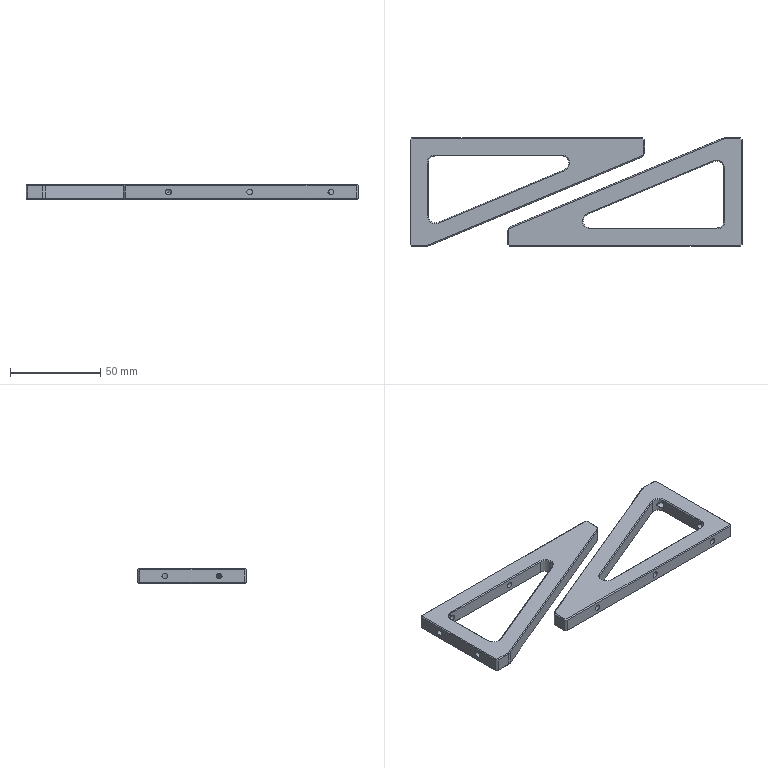CAM job | Mastercam | mm | 8 operations | part box 184.04 x 60 x 8
1. Contour (Ramp) | 6 - 6 平底刀
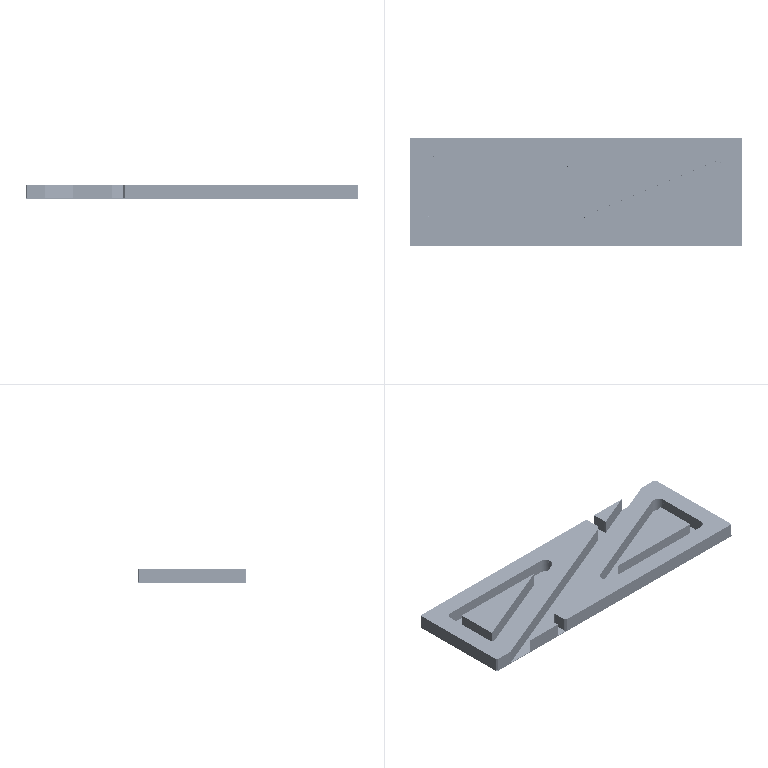2. Contour (2D) | 7 - 4 平底刀
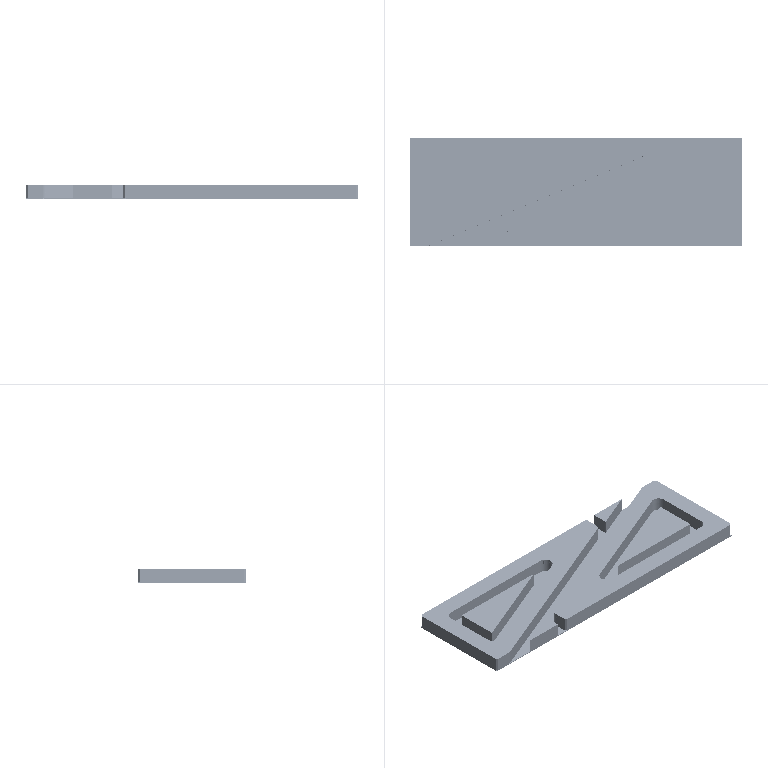3. Contour (2D chamfer) | 2 - 6定位倒角
4. Contour (2D) | 7 - 4 平底刀
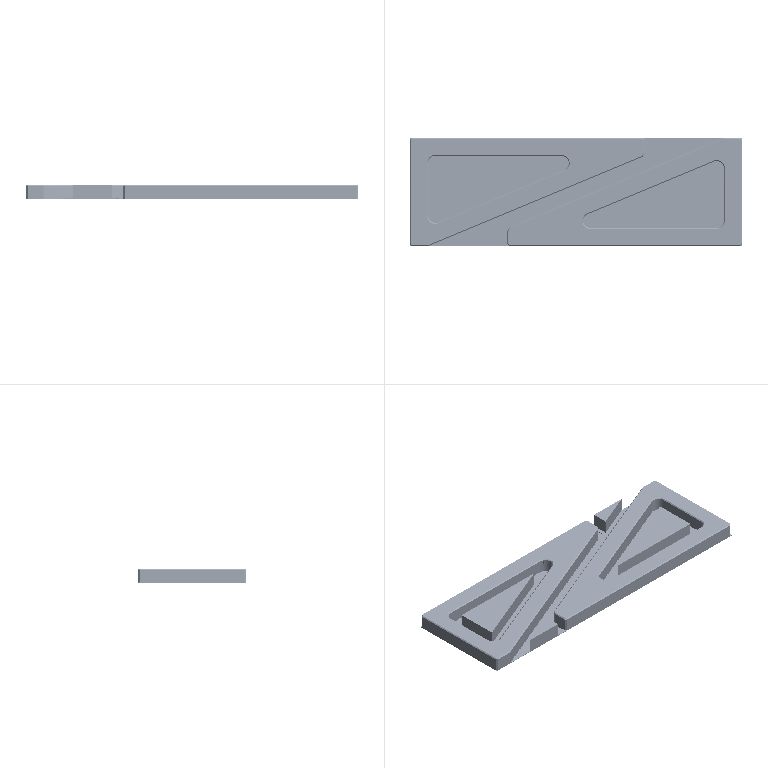5. Drill/Counterbore | 2 - 6定位倒角
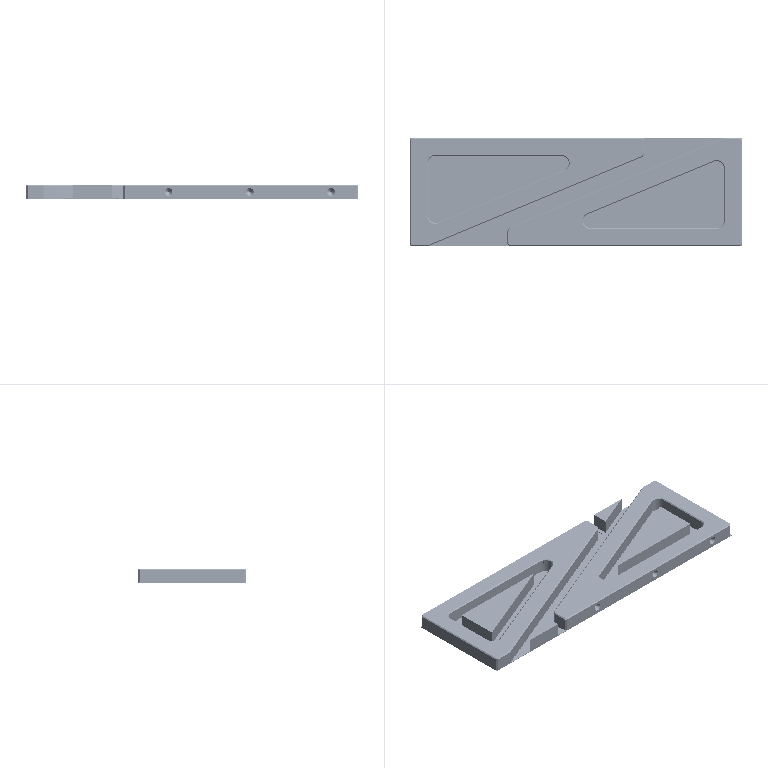6. Peck Drill | 12 - 3.3 钻头
7. Drill/Counterbore | 2 - 6定位倒角
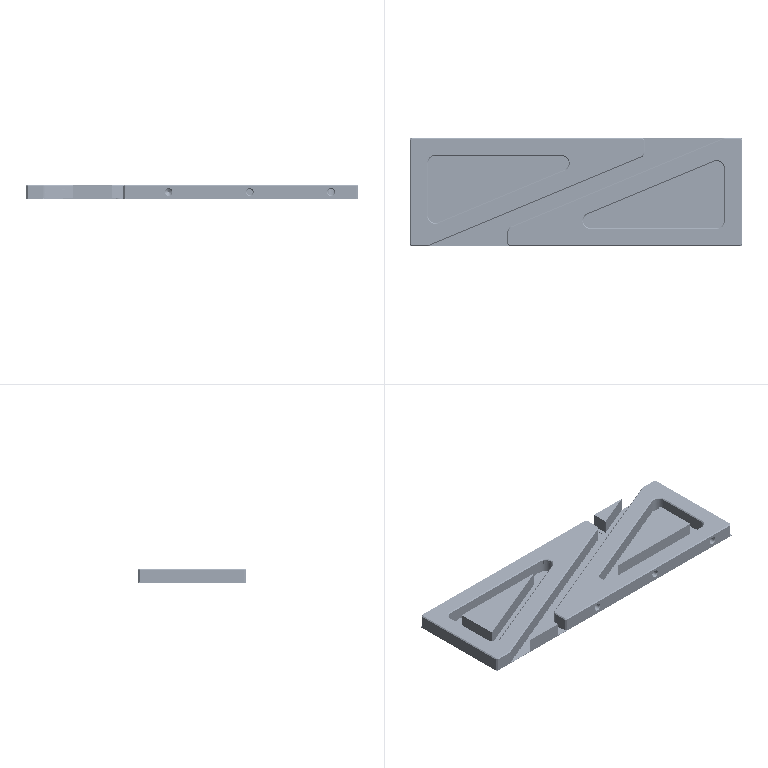8. Peck Drill | 12 - 3.3 钻头